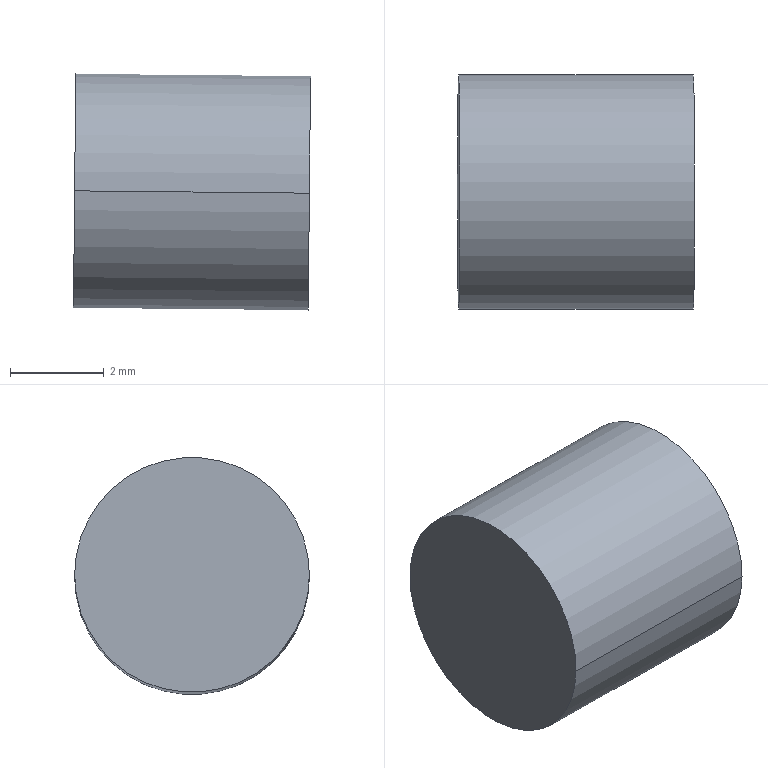Component | SolidWorks | Part7-1 | 1 solid | 10 faces | box 5.05 x 5 x 5.05 mm | volume 75 mm3 | cylinder 5 | plane 5 | commonest cylinder face diameters 1.7 x3 5 x2 | material 45
build123d program:
from build123d import *

# Parameters (mm, degrees)
SKETCH2_R                 = 2.5
BOSS_EXTRUDE1_DEPTH       = 5
SLOT_SERVOWIREENTRY_DEPTH = 3.1


with BuildPart() as part:
    # Sketch2 → Boss-Extrude1 (new body)
    with BuildSketch(Plane.XY):
        with Locations((0, -22.25)):
            Circle(SKETCH2_R)
    extrude(amount=BOSS_EXTRUDE1_DEPTH)

    # Sketch1 → Slot-ServoWireEntry (cut)
    with BuildSketch(Plane(origin=(0, 0, 0), x_dir=(-1, 0, 0), z_dir=(0, 0, -1))):
        with BuildLine():
            Line((-1.55, -21.387), (1.55, -21.387))
            ThreePointArc((1.55, -21.387), (2.4, -22.237), (1.55, -23.087))
            Line((1.55, -23.087), (-1.55, -23.087))
            ThreePointArc((-1.55, -23.087), (-2.4, -22.237), (-1.55, -21.387))
        make_face()
    extrude(amount=-SLOT_SERVOWIREENTRY_DEPTH, mode=Mode.SUBTRACT)


solid = part.part

# Placed as in the assembly
solid = solid.moved(Location((-19.564, 30.493, 6.846), (0, -89.439, -90)))
STEP:
#1=CARTESIAN_POINT('',(-0.9008,1.295,-0.6047));
#2=VERTEX_POINT('',#1);
#3=CARTESIAN_POINT('',(-0.9005,1.262,-0.5712));
#4=VERTEX_POINT('',#3);
#5=CARTESIAN_POINT('',(-0.9008,1.262,-0.6047));
#6=DIRECTION('',(1.,-0.,-0.009793));
#7=DIRECTION('',(0.,-1.,0.));
#8=AXIS2_PLACEMENT_3D('',#5,#6,#7);
#9=CIRCLE('',#8,0.03346);
#10=EDGE_CURVE('',#2,#4,#9,.T.);
#11=ORIENTED_EDGE('',*,*,#10,.F.);
#12=CARTESIAN_POINT('',(-0.7788,1.295,-0.6059));
#13=VERTEX_POINT('',#12);
#14=CARTESIAN_POINT('',(-0.9008,1.295,-0.6047));
#15=DIRECTION('',(1.,-0.,-0.009793));
#16=VECTOR('',#15,39.37);
#17=LINE('',#14,#16);
#18=EDGE_CURVE('',#2,#13,#17,.T.);
#19=ORIENTED_EDGE('',*,*,#18,.T.);
#20=CARTESIAN_POINT('',(-0.7785,1.262,-0.5724));
#21=VERTEX_POINT('',#20);
#22=CARTESIAN_POINT('',(-0.7788,1.262,-0.6059));
#23=DIRECTION('',(1.,-0.,-0.009793));
#24=DIRECTION('',(0.,-1.,0.));
#25=AXIS2_PLACEMENT_3D('',#22,#23,#24);
#26=CIRCLE('',#25,0.03346);
#27=EDGE_CURVE('',#13,#21,#26,.T.);
#28=ORIENTED_EDGE('',*,*,#27,.T.);
#29=CARTESIAN_POINT('',(-0.9005,1.262,-0.5712));
#30=DIRECTION('',(1.,-0.,-0.009793));
#31=VECTOR('',#30,39.37);
#32=LINE('',#29,#31);
#33=EDGE_CURVE('',#4,#21,#32,.T.);
#34=ORIENTED_EDGE('',*,*,#33,.F.);
#35=EDGE_LOOP('',(#11,#19,#28,#34));
#36=FACE_OUTER_BOUND('',#35,.T.);
#37=CARTESIAN_POINT('',(-0.9008,1.262,-0.6047));
#38=DIRECTION('',(1.,-0.,-0.009793));
#39=DIRECTION('',(0.,1.,0.));
#40=AXIS2_PLACEMENT_3D('',#37,#38,#39);
#41=CYLINDRICAL_SURFACE('',#40,0.03346);
#42=ADVANCED_FACE('',(#36),#41,.F.);
#43=CARTESIAN_POINT('',(-0.9756,1.102,-0.6045));
#44=VERTEX_POINT('',#43);
#45=CARTESIAN_POINT('',(-0.9756,1.299,-0.6045));
#46=VERTEX_POINT('',#45);
#47=CARTESIAN_POINT('',(-0.9756,1.201,-0.6045));
#48=DIRECTION('',(-1.,0.,0.009793));
#49=DIRECTION('',(0.,-1.,0.));
#50=AXIS2_PLACEMENT_3D('',#47,#48,#49);
#51=CIRCLE('',#50,0.09843);
#52=EDGE_CURVE('',#44,#46,#51,.T.);
#53=ORIENTED_EDGE('',*,*,#52,.F.);
#54=CARTESIAN_POINT('',(-0.7788,1.102,-0.6064));
#55=VERTEX_POINT('',#54);
#56=CARTESIAN_POINT('',(-0.9756,1.102,-0.6045));
#57=DIRECTION('',(1.,-0.,-0.009793));
#58=VECTOR('',#57,39.37);
#59=LINE('',#56,#58);
#60=EDGE_CURVE('',#44,#55,#59,.T.);
#61=ORIENTED_EDGE('',*,*,#60,.T.);
#62=CARTESIAN_POINT('',(-0.7788,1.299,-0.6064));
#63=VERTEX_POINT('',#62);
#64=CARTESIAN_POINT('',(-0.7788,1.201,-0.6064));
#65=DIRECTION('',(-1.,0.,0.009793));
#66=DIRECTION('',(0.,-1.,0.));
#67=AXIS2_PLACEMENT_3D('',#64,#65,#66);
#68=CIRCLE('',#67,0.09843);
#69=EDGE_CURVE('',#55,#63,#68,.T.);
#70=ORIENTED_EDGE('',*,*,#69,.T.);
#71=CARTESIAN_POINT('',(-0.9756,1.299,-0.6045));
#72=DIRECTION('',(1.,-0.,-0.009793));
#73=VECTOR('',#72,39.37);
#74=LINE('',#71,#73);
#75=EDGE_CURVE('',#46,#63,#74,.T.);
#76=ORIENTED_EDGE('',*,*,#75,.F.);
#77=EDGE_LOOP('',(#53,#61,#70,#76));
#78=FACE_OUTER_BOUND('',#77,.T.);
#79=CARTESIAN_POINT('',(-0.9756,1.201,-0.6045));
#80=DIRECTION('',(1.,-0.,-0.009793));
#81=DIRECTION('',(0.,1.,0.));
#82=AXIS2_PLACEMENT_3D('',#79,#80,#81);
#83=CYLINDRICAL_SURFACE('',#82,0.09843);
#84=ADVANCED_FACE('',(#78),#83,.T.);
#85=ORIENTED_EDGE('',*,*,#60,.F.);
#86=CARTESIAN_POINT('',(-0.9756,1.201,-0.6045));
#87=DIRECTION('',(-1.,0.,0.009793));
#88=DIRECTION('',(0.,-1.,0.));
#89=AXIS2_PLACEMENT_3D('',#86,#87,#88);
#90=CIRCLE('',#89,0.09843);
#91=EDGE_CURVE('',#46,#44,#90,.T.);
#92=ORIENTED_EDGE('',*,*,#91,.F.);
#93=ORIENTED_EDGE('',*,*,#75,.T.);
#94=CARTESIAN_POINT('',(-0.7788,1.201,-0.6064));
#95=DIRECTION('',(-1.,0.,0.009793));
#96=DIRECTION('',(0.,-1.,0.));
#97=AXIS2_PLACEMENT_3D('',#94,#95,#96);
#98=CIRCLE('',#97,0.09843);
#99=EDGE_CURVE('',#63,#55,#98,.T.);
#100=ORIENTED_EDGE('',*,*,#99,.T.);
#101=EDGE_LOOP('',(#85,#92,#93,#100));
#102=FACE_OUTER_BOUND('',#101,.T.);
#103=CARTESIAN_POINT('',(-0.9756,1.201,-0.6045));
#104=DIRECTION('',(1.,-0.,-0.009793));
#105=DIRECTION('',(0.,1.,0.));
#106=AXIS2_PLACEMENT_3D('',#103,#104,#105);
#107=CYLINDRICAL_SURFACE('',#106,0.09843);
#108=ADVANCED_FACE('',(#102),#107,.T.);
#109=ORIENTED_EDGE('',*,*,#91,.T.);
#110=ORIENTED_EDGE('',*,*,#52,.T.);
#111=EDGE_LOOP('',(#109,#110));
#112=FACE_OUTER_BOUND('',#111,.T.);
#113=CARTESIAN_POINT('',(-0.9756,1.201,-0.6045));
#114=DIRECTION('',(-1.,0.,0.009793));
#115=DIRECTION('',(-0.,-1.,-0.));
#116=AXIS2_PLACEMENT_3D('',#113,#114,#115);
#117=PLANE('',#116);
#118=ADVANCED_FACE('',(#112),#117,.T.);
#119=CARTESIAN_POINT('',(-0.7791,1.14,-0.6394));
#120=VERTEX_POINT('',#119);
#121=CARTESIAN_POINT('',(-0.7791,1.262,-0.6394));
#122=VERTEX_POINT('',#121);
#123=CARTESIAN_POINT('',(-0.7791,1.14,-0.6394));
#124=DIRECTION('',(0.,1.,0.));
#125=VECTOR('',#124,39.37);
#126=LINE('',#123,#125);
#127=EDGE_CURVE('',#120,#122,#126,.T.);
#128=ORIENTED_EDGE('',*,*,#127,.F.);
#129=CARTESIAN_POINT('',(-0.7785,1.14,-0.5724));
#130=VERTEX_POINT('',#129);
#131=CARTESIAN_POINT('',(-0.7788,1.14,-0.6059));
#132=DIRECTION('',(1.,-0.,-0.009793));
#133=DIRECTION('',(0.,1.,0.));
#134=AXIS2_PLACEMENT_3D('',#131,#132,#133);
#135=CIRCLE('',#134,0.03346);
#136=EDGE_CURVE('',#130,#120,#135,.T.);
#137=ORIENTED_EDGE('',*,*,#136,.F.);
#138=CARTESIAN_POINT('',(-0.7785,1.14,-0.5724));
#139=DIRECTION('',(-0.,-1.,-0.));
#140=VECTOR('',#139,39.37);
#141=LINE('',#138,#140);
#142=EDGE_CURVE('',#21,#130,#141,.T.);
#143=ORIENTED_EDGE('',*,*,#142,.F.);
#144=ORIENTED_EDGE('',*,*,#27,.F.);
#145=CARTESIAN_POINT('',(-0.7788,1.262,-0.6059));
#146=DIRECTION('',(1.,-0.,-0.009793));
#147=DIRECTION('',(0.,-1.,0.));
#148=AXIS2_PLACEMENT_3D('',#145,#146,#147);
#149=CIRCLE('',#148,0.03346);
#150=EDGE_CURVE('',#122,#13,#149,.T.);
#151=ORIENTED_EDGE('',*,*,#150,.F.);
#152=EDGE_LOOP('',(#128,#137,#143,#144,#151));
#153=FACE_BOUND('',#152,.T.);
#154=ORIENTED_EDGE('',*,*,#99,.F.);
#155=ORIENTED_EDGE('',*,*,#69,.F.);
#156=EDGE_LOOP('',(#154,#155));
#157=FACE_OUTER_BOUND('',#156,.T.);
#158=CARTESIAN_POINT('',(-0.7788,1.201,-0.6064));
#159=DIRECTION('',(-1.,0.,0.009793));
#160=DIRECTION('',(-0.,-1.,-0.));
#161=AXIS2_PLACEMENT_3D('',#158,#159,#160);
#162=PLANE('',#161);
#163=ADVANCED_FACE('',(#153,#157),#162,.F.);
#164=ORIENTED_EDGE('',*,*,#136,.T.);
#165=CARTESIAN_POINT('',(-0.9012,1.14,-0.6382));
#166=VERTEX_POINT('',#165);
#167=CARTESIAN_POINT('',(-0.9012,1.14,-0.6382));
#168=DIRECTION('',(1.,-0.,-0.009793));
#169=VECTOR('',#168,39.37);
#170=LINE('',#167,#169);
#171=EDGE_CURVE('',#166,#120,#170,.T.);
#172=ORIENTED_EDGE('',*,*,#171,.F.);
#173=CARTESIAN_POINT('',(-0.9005,1.14,-0.5712));
#174=VERTEX_POINT('',#173);
#175=CARTESIAN_POINT('',(-0.9008,1.14,-0.6047));
#176=DIRECTION('',(1.,-0.,-0.009793));
#177=DIRECTION('',(0.,1.,0.));
#178=AXIS2_PLACEMENT_3D('',#175,#176,#177);
#179=CIRCLE('',#178,0.03346);
#180=EDGE_CURVE('',#174,#166,#179,.T.);
#181=ORIENTED_EDGE('',*,*,#180,.F.);
#182=CARTESIAN_POINT('',(-0.9005,1.14,-0.5712));
#183=DIRECTION('',(1.,-0.,-0.009793));
#184=VECTOR('',#183,39.37);
#185=LINE('',#182,#184);
#186=EDGE_CURVE('',#174,#130,#185,.T.);
#187=ORIENTED_EDGE('',*,*,#186,.T.);
#188=EDGE_LOOP('',(#164,#172,#181,#187));
#189=FACE_OUTER_BOUND('',#188,.T.);
#190=CARTESIAN_POINT('',(-0.9008,1.14,-0.6047));
#191=DIRECTION('',(1.,-0.,-0.009793));
#192=DIRECTION('',(0.,1.,0.));
#193=AXIS2_PLACEMENT_3D('',#190,#191,#192);
#194=CYLINDRICAL_SURFACE('',#193,0.03346);
#195=ADVANCED_FACE('',(#189),#194,.F.);
#196=ORIENTED_EDGE('',*,*,#142,.T.);
#197=ORIENTED_EDGE('',*,*,#186,.F.);
#198=CARTESIAN_POINT('',(-0.9005,1.14,-0.5712));
#199=DIRECTION('',(-0.,-1.,-0.));
#200=VECTOR('',#199,39.37);
#201=LINE('',#198,#200);
#202=EDGE_CURVE('',#4,#174,#201,.T.);
#203=ORIENTED_EDGE('',*,*,#202,.F.);
#204=ORIENTED_EDGE('',*,*,#33,.T.);
#205=EDGE_LOOP('',(#196,#197,#203,#204));
#206=FACE_OUTER_BOUND('',#205,.T.);
#207=CARTESIAN_POINT('',(-0.9005,1.14,-0.5712));
#208=DIRECTION('',(0.009793,-0.,1.));
#209=DIRECTION('',(-1.,0.,0.009793));
#210=AXIS2_PLACEMENT_3D('',#207,#208,#209);
#211=PLANE('',#210);
#212=ADVANCED_FACE('',(#206),#211,.F.);
#213=ORIENTED_EDGE('',*,*,#18,.F.);
#214=CARTESIAN_POINT('',(-0.9012,1.262,-0.6382));
#215=VERTEX_POINT('',#214);
#216=CARTESIAN_POINT('',(-0.9008,1.262,-0.6047));
#217=DIRECTION('',(1.,-0.,-0.009793));
#218=DIRECTION('',(0.,-1.,0.));
#219=AXIS2_PLACEMENT_3D('',#216,#217,#218);
#220=CIRCLE('',#219,0.03346);
#221=EDGE_CURVE('',#215,#2,#220,.T.);
#222=ORIENTED_EDGE('',*,*,#221,.F.);
#223=CARTESIAN_POINT('',(-0.9012,1.262,-0.6382));
#224=DIRECTION('',(1.,-0.,-0.009793));
#225=VECTOR('',#224,39.37);
#226=LINE('',#223,#225);
#227=EDGE_CURVE('',#215,#122,#226,.T.);
#228=ORIENTED_EDGE('',*,*,#227,.T.);
#229=ORIENTED_EDGE('',*,*,#150,.T.);
#230=EDGE_LOOP('',(#213,#222,#228,#229));
#231=FACE_OUTER_BOUND('',#230,.T.);
#232=CARTESIAN_POINT('',(-0.9008,1.262,-0.6047));
#233=DIRECTION('',(1.,-0.,-0.009793));
#234=DIRECTION('',(0.,1.,0.));
#235=AXIS2_PLACEMENT_3D('',#232,#233,#234);
#236=CYLINDRICAL_SURFACE('',#235,0.03346);
#237=ADVANCED_FACE('',(#231),#236,.F.);
#238=ORIENTED_EDGE('',*,*,#127,.T.);
#239=ORIENTED_EDGE('',*,*,#227,.F.);
#240=CARTESIAN_POINT('',(-0.9012,1.14,-0.6382));
#241=DIRECTION('',(0.,1.,0.));
#242=VECTOR('',#241,39.37);
#243=LINE('',#240,#242);
#244=EDGE_CURVE('',#166,#215,#243,.T.);
#245=ORIENTED_EDGE('',*,*,#244,.F.);
#246=ORIENTED_EDGE('',*,*,#171,.T.);
#247=EDGE_LOOP('',(#238,#239,#245,#246));
#248=FACE_OUTER_BOUND('',#247,.T.);
#249=CARTESIAN_POINT('',(-0.9012,1.14,-0.6382));
#250=DIRECTION('',(-0.009793,0.,-1.));
#251=DIRECTION('',(1.,-0.,-0.009793));
#252=AXIS2_PLACEMENT_3D('',#249,#250,#251);
#253=PLANE('',#252);
#254=ADVANCED_FACE('',(#248),#253,.F.);
#255=ORIENTED_EDGE('',*,*,#180,.T.);
#256=ORIENTED_EDGE('',*,*,#244,.T.);
#257=ORIENTED_EDGE('',*,*,#221,.T.);
#258=ORIENTED_EDGE('',*,*,#10,.T.);
#259=ORIENTED_EDGE('',*,*,#202,.T.);
#260=EDGE_LOOP('',(#255,#256,#257,#258,#259));
#261=FACE_OUTER_BOUND('',#260,.T.);
#262=CARTESIAN_POINT('',(-0.9008,1.14,-0.6047));
#263=DIRECTION('',(1.,-0.,-0.009793));
#264=DIRECTION('',(0.,1.,0.));
#265=AXIS2_PLACEMENT_3D('',#262,#263,#264);
#266=PLANE('',#265);
#267=ADVANCED_FACE('',(#261),#266,.T.);
#268=CLOSED_SHELL('',(#42,#84,#108,#118,#163,#195,#212,#237,#254,#267));
#269=MANIFOLD_SOLID_BREP('',#268);
#270=CARTESIAN_POINT('',(0.,0.,0.));
#271=DIRECTION('',(0.,0.,1.));
#272=DIRECTION('',(1.,0.,0.));
#273=AXIS2_PLACEMENT_3D('',#270,#271,#272);
#274=(LENGTH_UNIT()NAMED_UNIT(*)SI_UNIT($,.METRE.));
#275=LENGTH_MEASURE_WITH_UNIT(LENGTH_MEASURE(0.0254),#274);
#276=DIMENSIONAL_EXPONENTS(1.,0.,0.,0.,0.,0.,0.);
#277=(CONVERSION_BASED_UNIT('',#275)LENGTH_UNIT()NAMED_UNIT(#276));
#278=UNCERTAINTY_MEASURE_WITH_UNIT(LENGTH_MEASURE(0.00001),#277,'','');
#279=(NAMED_UNIT(*)PLANE_ANGLE_UNIT()SI_UNIT($,.RADIAN.));
#280=(NAMED_UNIT(*)SI_UNIT($,.STERADIAN.)SOLID_ANGLE_UNIT());
#281=(GEOMETRIC_REPRESENTATION_CONTEXT(3)GLOBAL_UNCERTAINTY_ASSIGNED_CONTEXT((#278))GLOBAL_UNIT_ASSIGNED_CONTEXT((#277,#279,#280))REPRESENTATION_CONTEXT('',''));
#282=ADVANCED_BREP_SHAPE_REPRESENTATION('',(#269,#273),#281);
#283=COLOUR_RGB('',0.7922,0.8196,0.9333);
#284=FILL_AREA_STYLE_COLOUR('',#283);
#285=FILL_AREA_STYLE('',(#284));
#286=SURFACE_STYLE_FILL_AREA(#285);
#287=SURFACE_SIDE_STYLE('',(#286));
#288=SURFACE_STYLE_USAGE(.BOTH.,#287);
#289=PRESENTATION_STYLE_ASSIGNMENT((#288));
#290=STYLED_ITEM('',(#289),#269);
#291=(LENGTH_UNIT()NAMED_UNIT(*)SI_UNIT($,.METRE.));
#292=LENGTH_MEASURE_WITH_UNIT(LENGTH_MEASURE(0.0254),#291);
#293=DIMENSIONAL_EXPONENTS(1.,0.,0.,0.,0.,0.,0.);
#294=(CONVERSION_BASED_UNIT('',#292)LENGTH_UNIT()NAMED_UNIT(#293));
#295=UNCERTAINTY_MEASURE_WITH_UNIT(LENGTH_MEASURE(0.00001),#294,'','');
#296=(NAMED_UNIT(*)PLANE_ANGLE_UNIT()SI_UNIT($,.RADIAN.));
#297=(NAMED_UNIT(*)SI_UNIT($,.STERADIAN.)SOLID_ANGLE_UNIT());
#298=(GEOMETRIC_REPRESENTATION_CONTEXT(3)GLOBAL_UNCERTAINTY_ASSIGNED_CONTEXT((#295))GLOBAL_UNIT_ASSIGNED_CONTEXT((#294,#296,#297))REPRESENTATION_CONTEXT('',''));
#299=MECHANICAL_DESIGN_GEOMETRIC_PRESENTATION_REPRESENTATION('',(#290),#298);
#300=PRESENTATION_LAYER_ASSIGNMENT('','',(#290));